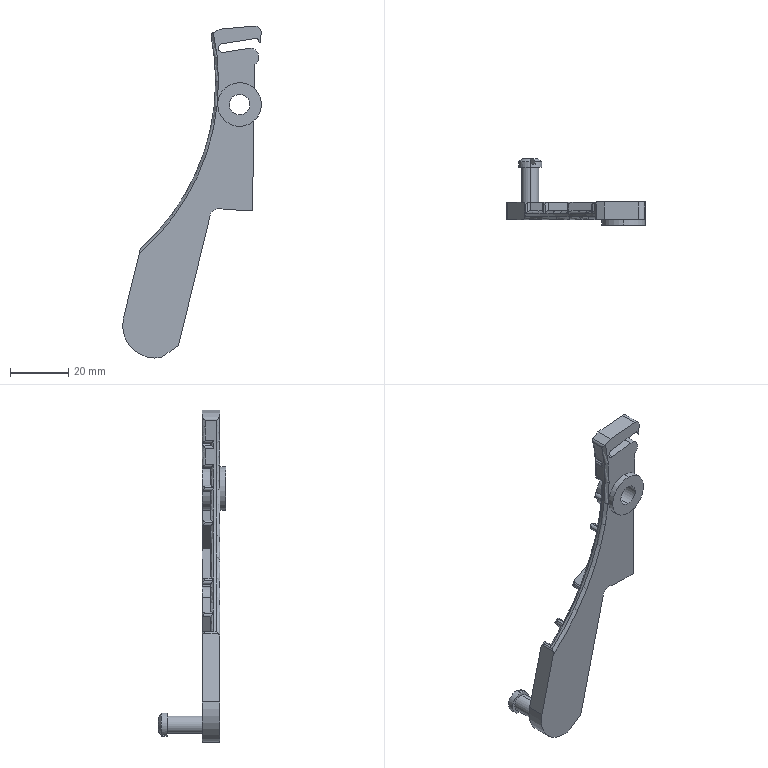Component | SolidWorks | ReversingArm-101 | 1 solid | 115 faces | volume 9101 mm3 | plane 54 | cylinder 44 | torus 14 | cone 3 | commonest cylinder face diameters 2 x23 15 x6 6 x4 8 x2 10 x2 22.183 x2 7 x2 3 x1